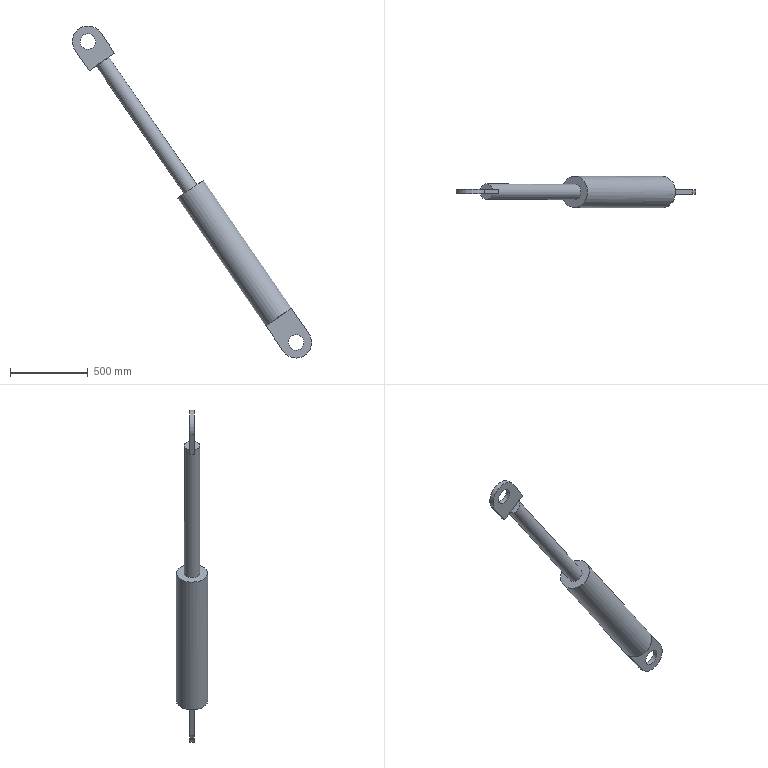Component | NX | YEYAGANG | 2 solids | 21 faces | volume 42607863 mm3 | plane 15 | cylinder 6 | commonest cylinder face diameters 100 x3 200 x2 202.237 x1